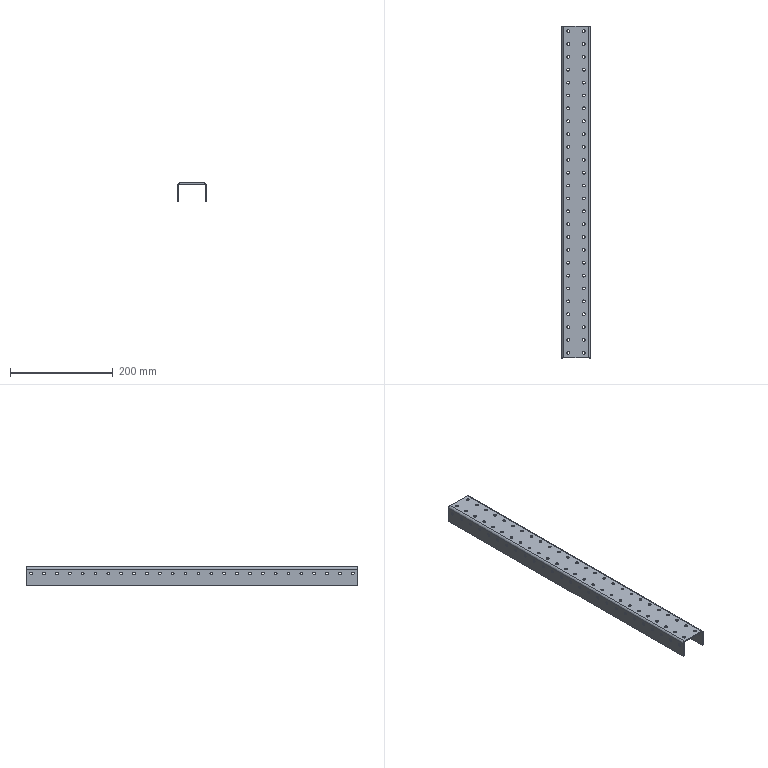Component | SolidWorks | BottomPlateMiddleBeam-1 | 1 solid | 238 faces | volume 147995 mm3 | cylinder 212 | plane 26 | commonest cylinder face diameters 5.4 x208 8 x2 4 x2